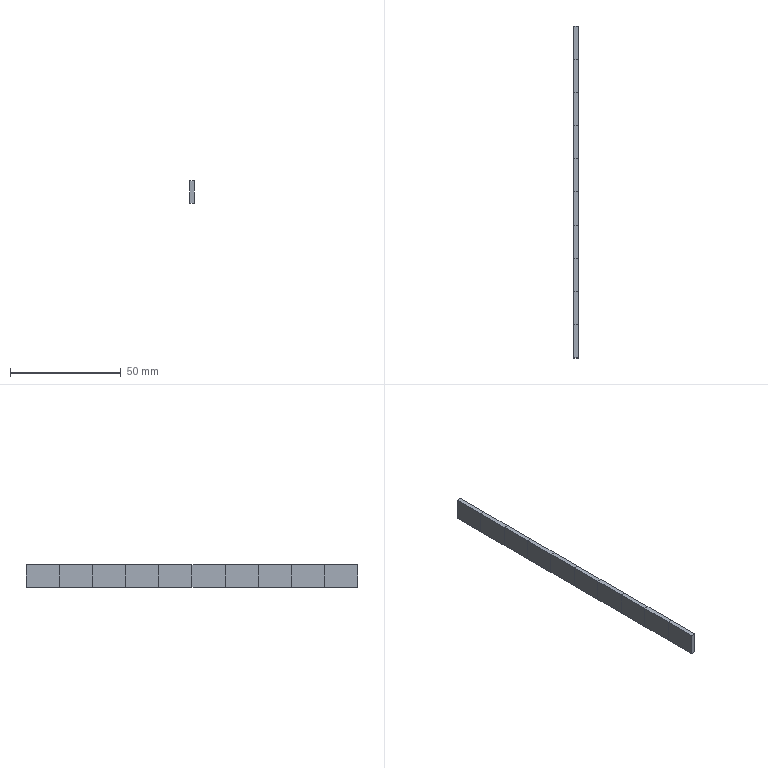Component | NX | 12_SINKBODY | 10 solids | 60 faces | volume 3000 mm3 | plane 60